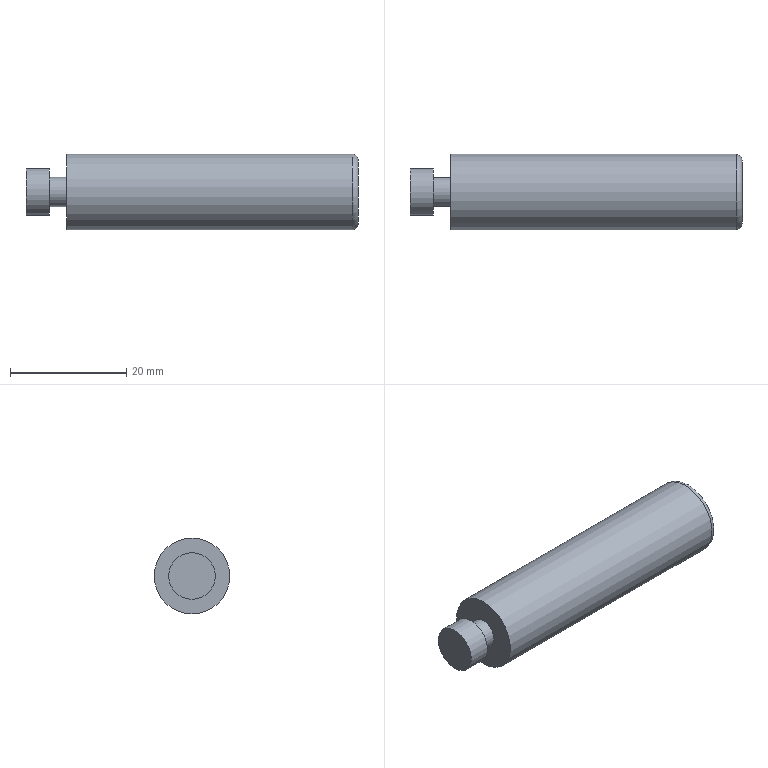Component | NX | SHAFT_02 | 1 solid | 8 faces | box 57 x 13 x 13 mm | volume 6888 mm3 | plane 4 | cylinder 3 | torus 1 | commonest cylinder face diameters 8 x1 5 x1 13 x1
STEP:
#1=CARTESIAN_POINT('',(0.,0.,0.));
#2=DIRECTION('',(0.,0.,1.));
#3=DIRECTION('',(1.,0.,0.));
#4=AXIS2_PLACEMENT_3D('',#1,#2,#3);
#5=CARTESIAN_POINT('',(100.,3.,1.5));
#6=VERTEX_POINT('',#5);
#7=CARTESIAN_POINT('',(100.,3.,4.));
#8=DIRECTION('',(1.,0.,0.));
#9=DIRECTION('',(0.,0.,-1.));
#10=AXIS2_PLACEMENT_3D('',#7,#8,#9);
#11=CIRCLE('',#10,2.5);
#12=CARTESIAN_POINT('',(100.,3.,4.));
#13=DIRECTION('',(1.,0.,0.));
#14=DIRECTION('',(0.,0.,-1.));
#15=AXIS2_PLACEMENT_3D('',#12,#13,#14);
#16=PLANE('',#15);
#17=CARTESIAN_POINT('',(0.,0.));
#18=DIRECTION('',(1.,0.));
#19=AXIS2_PLACEMENT_2D('',#17,#18);
#20=CIRCLE('',#19,2.5);
#21=(GEOMETRIC_REPRESENTATION_CONTEXT(2)PARAMETRIC_REPRESENTATION_CONTEXT()REPRESENTATION_CONTEXT('',''));
#22=DEFINITIONAL_REPRESENTATION('',(#20),#21);
#23=PCURVE('',#16,#22);
#24=CARTESIAN_POINT('',(100.,3.,4.));
#25=DIRECTION('',(1.,0.,0.));
#26=DIRECTION('',(0.,0.,-1.));
#27=AXIS2_PLACEMENT_3D('',#24,#25,#26);
#28=CYLINDRICAL_SURFACE('',#27,2.5);
#29=CARTESIAN_POINT('',(0.,0.));
#30=DIRECTION('',(1.,0.));
#31=VECTOR('',#30,1.);
#32=LINE('',#29,#31);
#33=(GEOMETRIC_REPRESENTATION_CONTEXT(2)PARAMETRIC_REPRESENTATION_CONTEXT()REPRESENTATION_CONTEXT('',''));
#34=DEFINITIONAL_REPRESENTATION('',(#32),#33);
#35=PCURVE('',#28,#34);
#36=SURFACE_CURVE('',#11,(#23,#35),.PCURVE_S1.);
#37=EDGE_CURVE('',#6,#6,#36,.T.);
#38=ORIENTED_EDGE('',*,*,#37,.F.);
#39=EDGE_LOOP('',(#38));
#40=FACE_BOUND('',#39,.T.);
#41=CARTESIAN_POINT('',(100.,3.,0.));
#42=VERTEX_POINT('',#41);
#43=CARTESIAN_POINT('',(100.,3.,4.));
#44=DIRECTION('',(-1.,0.,0.));
#45=DIRECTION('',(0.,0.,-1.));
#46=AXIS2_PLACEMENT_3D('',#43,#44,#45);
#47=CIRCLE('',#46,4.);
#48=CARTESIAN_POINT('',(4.,0.));
#49=CARTESIAN_POINT('',(4.,-6.928));
#50=CARTESIAN_POINT('',(-2.,-3.464));
#51=CARTESIAN_POINT('',(-8.,-0.));
#52=CARTESIAN_POINT('',(-2.,3.464));
#53=CARTESIAN_POINT('',(4.,6.928));
#54=CARTESIAN_POINT('',(4.,0.));
#55=(BOUNDED_CURVE()B_SPLINE_CURVE(2,(#48,#49,#50,#51,#52,#53,#54),.UNSPECIFIED.,.T.,.F.)B_SPLINE_CURVE_WITH_KNOTS((1,2,2,2,2,1),(-2.094,0.,2.094,4.189,6.283,8.378),.UNSPECIFIED.)CURVE()GEOMETRIC_REPRESENTATION_ITEM()RATIONAL_B_SPLINE_CURVE((1.,0.5,1.,0.5,1.,0.5,1.))REPRESENTATION_ITEM(''));
#56=(GEOMETRIC_REPRESENTATION_CONTEXT(2)PARAMETRIC_REPRESENTATION_CONTEXT()REPRESENTATION_CONTEXT('',''));
#57=DEFINITIONAL_REPRESENTATION('',(#55),#56);
#58=PCURVE('',#16,#57);
#59=CARTESIAN_POINT('',(96.,3.,4.));
#60=DIRECTION('',(1.,0.,0.));
#61=DIRECTION('',(0.,0.,-1.));
#62=AXIS2_PLACEMENT_3D('',#59,#60,#61);
#63=CYLINDRICAL_SURFACE('',#62,4.);
#64=CARTESIAN_POINT('',(6.283,4.));
#65=DIRECTION('',(-1.,0.));
#66=VECTOR('',#65,1.);
#67=LINE('',#64,#66);
#68=(GEOMETRIC_REPRESENTATION_CONTEXT(2)PARAMETRIC_REPRESENTATION_CONTEXT()REPRESENTATION_CONTEXT('',''));
#69=DEFINITIONAL_REPRESENTATION('',(#67),#68);
#70=PCURVE('',#63,#69);
#71=SURFACE_CURVE('',#47,(#58,#70),.PCURVE_S1.);
#72=EDGE_CURVE('',#42,#42,#71,.T.);
#73=ORIENTED_EDGE('',*,*,#72,.F.);
#74=EDGE_LOOP('',(#73));
#75=FACE_BOUND('',#74,.T.);
#76=ADVANCED_FACE('',(#40,#75),#16,.T.);
#77=CARTESIAN_POINT('',(96.,3.,0.));
#78=VERTEX_POINT('',#77);
#79=CARTESIAN_POINT('',(96.,3.,4.));
#80=DIRECTION('',(1.,0.,0.));
#81=DIRECTION('',(0.,0.,-1.));
#82=AXIS2_PLACEMENT_3D('',#79,#80,#81);
#83=CIRCLE('',#82,4.);
#84=CARTESIAN_POINT('',(96.,3.,4.));
#85=DIRECTION('',(-1.,0.,0.));
#86=DIRECTION('',(0.,0.,1.));
#87=AXIS2_PLACEMENT_3D('',#84,#85,#86);
#88=PLANE('',#87);
#89=CARTESIAN_POINT('',(-4.,0.));
#90=CARTESIAN_POINT('',(-4.,6.928));
#91=CARTESIAN_POINT('',(2.,3.464));
#92=CARTESIAN_POINT('',(8.,0.));
#93=CARTESIAN_POINT('',(2.,-3.464));
#94=CARTESIAN_POINT('',(-4.,-6.928));
#95=CARTESIAN_POINT('',(-4.,0.));
#96=(BOUNDED_CURVE()B_SPLINE_CURVE(2,(#89,#90,#91,#92,#93,#94,#95),.UNSPECIFIED.,.T.,.F.)B_SPLINE_CURVE_WITH_KNOTS((1,2,2,2,2,1),(-2.094,0.,2.094,4.189,6.283,8.378),.UNSPECIFIED.)CURVE()GEOMETRIC_REPRESENTATION_ITEM()RATIONAL_B_SPLINE_CURVE((1.,0.5,1.,0.5,1.,0.5,1.))REPRESENTATION_ITEM(''));
#97=(GEOMETRIC_REPRESENTATION_CONTEXT(2)PARAMETRIC_REPRESENTATION_CONTEXT()REPRESENTATION_CONTEXT('',''));
#98=DEFINITIONAL_REPRESENTATION('',(#96),#97);
#99=PCURVE('',#88,#98);
#100=CARTESIAN_POINT('',(0.,0.));
#101=DIRECTION('',(1.,0.));
#102=VECTOR('',#101,1.);
#103=LINE('',#100,#102);
#104=(GEOMETRIC_REPRESENTATION_CONTEXT(2)PARAMETRIC_REPRESENTATION_CONTEXT()REPRESENTATION_CONTEXT('',''));
#105=DEFINITIONAL_REPRESENTATION('',(#103),#104);
#106=PCURVE('',#63,#105);
#107=SURFACE_CURVE('',#83,(#99,#106),.PCURVE_S1.);
#108=EDGE_CURVE('',#78,#78,#107,.T.);
#109=ORIENTED_EDGE('',*,*,#108,.F.);
#110=EDGE_LOOP('',(#109));
#111=FACE_BOUND('',#110,.T.);
#112=ADVANCED_FACE('',(#111),#88,.T.);
#113=ORIENTED_EDGE('',*,*,#72,.T.);
#114=CARTESIAN_POINT('',(96.,3.,0.));
#115=CARTESIAN_POINT('',(100.,3.,0.));
#116=B_SPLINE_CURVE_WITH_KNOTS('',1,(#114,#115),.UNSPECIFIED.,.F.,.F.,(2,2),(0.,4.),.PIECEWISE_BEZIER_KNOTS.);
#117=CARTESIAN_POINT('',(0.,0.));
#118=DIRECTION('',(0.,1.));
#119=VECTOR('',#118,1.);
#120=LINE('',#117,#119);
#121=(GEOMETRIC_REPRESENTATION_CONTEXT(2)PARAMETRIC_REPRESENTATION_CONTEXT()REPRESENTATION_CONTEXT('',''));
#122=DEFINITIONAL_REPRESENTATION('',(#120),#121);
#123=PCURVE('',#63,#122);
#124=CARTESIAN_POINT('',(6.283,0.));
#125=DIRECTION('',(0.,1.));
#126=VECTOR('',#125,1.);
#127=LINE('',#124,#126);
#128=(GEOMETRIC_REPRESENTATION_CONTEXT(2)PARAMETRIC_REPRESENTATION_CONTEXT()REPRESENTATION_CONTEXT('',''));
#129=DEFINITIONAL_REPRESENTATION('',(#127),#128);
#130=PCURVE('',#63,#129);
#131=SEAM_CURVE('',#116,(#123,#130),.PCURVE_S1.);
#132=EDGE_CURVE('',#78,#42,#131,.T.);
#133=ORIENTED_EDGE('',*,*,#132,.F.);
#134=ORIENTED_EDGE('',*,*,#108,.T.);
#135=ORIENTED_EDGE('',*,*,#132,.T.);
#136=EDGE_LOOP('',(#113,#133,#134,#135));
#137=FACE_BOUND('',#136,.T.);
#138=ADVANCED_FACE('',(#137),#63,.T.);
#139=CARTESIAN_POINT('',(103.,3.,1.5));
#140=VERTEX_POINT('',#139);
#141=CARTESIAN_POINT('',(103.,3.,4.));
#142=DIRECTION('',(-1.,0.,0.));
#143=DIRECTION('',(0.,0.,-1.));
#144=AXIS2_PLACEMENT_3D('',#141,#142,#143);
#145=CIRCLE('',#144,2.5);
#146=CARTESIAN_POINT('',(6.283,3.));
#147=DIRECTION('',(-1.,0.));
#148=VECTOR('',#147,1.);
#149=LINE('',#146,#148);
#150=(GEOMETRIC_REPRESENTATION_CONTEXT(2)PARAMETRIC_REPRESENTATION_CONTEXT()REPRESENTATION_CONTEXT('',''));
#151=DEFINITIONAL_REPRESENTATION('',(#149),#150);
#152=PCURVE('',#28,#151);
#153=CARTESIAN_POINT('',(103.,3.,4.));
#154=DIRECTION('',(-1.,0.,0.));
#155=DIRECTION('',(0.,0.,1.));
#156=AXIS2_PLACEMENT_3D('',#153,#154,#155);
#157=PLANE('',#156);
#158=CARTESIAN_POINT('',(0.,0.));
#159=DIRECTION('',(-1.,0.));
#160=AXIS2_PLACEMENT_2D('',#158,#159);
#161=CIRCLE('',#160,2.5);
#162=(GEOMETRIC_REPRESENTATION_CONTEXT(2)PARAMETRIC_REPRESENTATION_CONTEXT()REPRESENTATION_CONTEXT('',''));
#163=DEFINITIONAL_REPRESENTATION('',(#161),#162);
#164=PCURVE('',#157,#163);
#165=SURFACE_CURVE('',#145,(#152,#164),.PCURVE_S1.);
#166=EDGE_CURVE('',#140,#140,#165,.T.);
#167=ORIENTED_EDGE('',*,*,#166,.T.);
#168=CARTESIAN_POINT('',(100.,3.,1.5));
#169=CARTESIAN_POINT('',(103.,3.,1.5));
#170=B_SPLINE_CURVE_WITH_KNOTS('',1,(#168,#169),.UNSPECIFIED.,.F.,.F.,(2,2),(0.,3.),.PIECEWISE_BEZIER_KNOTS.);
#171=CARTESIAN_POINT('',(0.,0.));
#172=DIRECTION('',(0.,1.));
#173=VECTOR('',#172,1.);
#174=LINE('',#171,#173);
#175=(GEOMETRIC_REPRESENTATION_CONTEXT(2)PARAMETRIC_REPRESENTATION_CONTEXT()REPRESENTATION_CONTEXT('',''));
#176=DEFINITIONAL_REPRESENTATION('',(#174),#175);
#177=PCURVE('',#28,#176);
#178=CARTESIAN_POINT('',(6.283,0.));
#179=DIRECTION('',(0.,1.));
#180=VECTOR('',#179,1.);
#181=LINE('',#178,#180);
#182=(GEOMETRIC_REPRESENTATION_CONTEXT(2)PARAMETRIC_REPRESENTATION_CONTEXT()REPRESENTATION_CONTEXT('',''));
#183=DEFINITIONAL_REPRESENTATION('',(#181),#182);
#184=PCURVE('',#28,#183);
#185=SEAM_CURVE('',#170,(#177,#184),.PCURVE_S1.);
#186=EDGE_CURVE('',#6,#140,#185,.T.);
#187=ORIENTED_EDGE('',*,*,#186,.F.);
#188=ORIENTED_EDGE('',*,*,#37,.T.);
#189=ORIENTED_EDGE('',*,*,#186,.T.);
#190=EDGE_LOOP('',(#167,#187,#188,#189));
#191=FACE_BOUND('',#190,.T.);
#192=ADVANCED_FACE('',(#191),#28,.T.);
#193=CARTESIAN_POINT('',(153.,3.,-1.5));
#194=VERTEX_POINT('',#193);
#195=CARTESIAN_POINT('',(153.,3.,4.));
#196=DIRECTION('',(1.,0.,0.));
#197=DIRECTION('',(0.,0.,-1.));
#198=AXIS2_PLACEMENT_3D('',#195,#196,#197);
#199=CIRCLE('',#198,5.5);
#200=CARTESIAN_POINT('',(153.,3.,4.));
#201=DIRECTION('',(1.,0.,0.));
#202=DIRECTION('',(0.,0.,-1.));
#203=AXIS2_PLACEMENT_3D('',#200,#201,#202);
#204=PLANE('',#203);
#205=CARTESIAN_POINT('',(0.,0.));
#206=DIRECTION('',(1.,0.));
#207=AXIS2_PLACEMENT_2D('',#205,#206);
#208=CIRCLE('',#207,5.5);
#209=(GEOMETRIC_REPRESENTATION_CONTEXT(2)PARAMETRIC_REPRESENTATION_CONTEXT()REPRESENTATION_CONTEXT('',''));
#210=DEFINITIONAL_REPRESENTATION('',(#208),#209);
#211=PCURVE('',#204,#210);
#212=CARTESIAN_POINT('',(152.,3.,4.));
#213=DIRECTION('',(1.,0.,0.));
#214=DIRECTION('',(0.,0.,-1.));
#215=AXIS2_PLACEMENT_3D('',#212,#213,#214);
#216=TOROIDAL_SURFACE('',#215,5.5,1.);
#217=CARTESIAN_POINT('',(0.,7.854));
#218=DIRECTION('',(1.,0.));
#219=VECTOR('',#218,1.);
#220=LINE('',#217,#219);
#221=(GEOMETRIC_REPRESENTATION_CONTEXT(2)PARAMETRIC_REPRESENTATION_CONTEXT()REPRESENTATION_CONTEXT('',''));
#222=DEFINITIONAL_REPRESENTATION('',(#220),#221);
#223=PCURVE('',#216,#222);
#224=SURFACE_CURVE('',#199,(#211,#223),.PCURVE_S1.);
#225=EDGE_CURVE('',#194,#194,#224,.T.);
#226=ORIENTED_EDGE('',*,*,#225,.T.);
#227=EDGE_LOOP('',(#226));
#228=FACE_BOUND('',#227,.T.);
#229=ADVANCED_FACE('',(#228),#204,.T.);
#230=ORIENTED_EDGE('',*,*,#166,.F.);
#231=EDGE_LOOP('',(#230));
#232=FACE_BOUND('',#231,.T.);
#233=CARTESIAN_POINT('',(103.,3.,-2.5));
#234=VERTEX_POINT('',#233);
#235=CARTESIAN_POINT('',(103.,3.,4.));
#236=DIRECTION('',(1.,0.,0.));
#237=DIRECTION('',(0.,0.,-1.));
#238=AXIS2_PLACEMENT_3D('',#235,#236,#237);
#239=CIRCLE('',#238,6.5);
#240=CARTESIAN_POINT('',(-6.5,0.));
#241=CARTESIAN_POINT('',(-6.5,11.258));
#242=CARTESIAN_POINT('',(3.25,5.629));
#243=CARTESIAN_POINT('',(13.,0.));
#244=CARTESIAN_POINT('',(3.25,-5.629));
#245=CARTESIAN_POINT('',(-6.5,-11.258));
#246=CARTESIAN_POINT('',(-6.5,0.));
#247=(BOUNDED_CURVE()B_SPLINE_CURVE(2,(#240,#241,#242,#243,#244,#245,#246),.UNSPECIFIED.,.T.,.F.)B_SPLINE_CURVE_WITH_KNOTS((1,2,2,2,2,1),(-2.094,0.,2.094,4.189,6.283,8.378),.UNSPECIFIED.)CURVE()GEOMETRIC_REPRESENTATION_ITEM()RATIONAL_B_SPLINE_CURVE((1.,0.5,1.,0.5,1.,0.5,1.))REPRESENTATION_ITEM(''));
#248=(GEOMETRIC_REPRESENTATION_CONTEXT(2)PARAMETRIC_REPRESENTATION_CONTEXT()REPRESENTATION_CONTEXT('',''));
#249=DEFINITIONAL_REPRESENTATION('',(#247),#248);
#250=PCURVE('',#157,#249);
#251=CARTESIAN_POINT('',(103.,3.,4.));
#252=DIRECTION('',(1.,0.,0.));
#253=DIRECTION('',(0.,0.,-1.));
#254=AXIS2_PLACEMENT_3D('',#251,#252,#253);
#255=CYLINDRICAL_SURFACE('',#254,6.5);
#256=CARTESIAN_POINT('',(0.,0.));
#257=DIRECTION('',(1.,0.));
#258=VECTOR('',#257,1.);
#259=LINE('',#256,#258);
#260=(GEOMETRIC_REPRESENTATION_CONTEXT(2)PARAMETRIC_REPRESENTATION_CONTEXT()REPRESENTATION_CONTEXT('',''));
#261=DEFINITIONAL_REPRESENTATION('',(#259),#260);
#262=PCURVE('',#255,#261);
#263=SURFACE_CURVE('',#239,(#250,#262),.PCURVE_S1.);
#264=EDGE_CURVE('',#234,#234,#263,.T.);
#265=ORIENTED_EDGE('',*,*,#264,.F.);
#266=EDGE_LOOP('',(#265));
#267=FACE_BOUND('',#266,.T.);
#268=ADVANCED_FACE('',(#232,#267),#157,.T.);
#269=CARTESIAN_POINT('',(152.,3.,-2.5));
#270=VERTEX_POINT('',#269);
#271=CARTESIAN_POINT('',(152.,3.,4.));
#272=DIRECTION('',(-1.,0.,0.));
#273=DIRECTION('',(0.,0.,-1.));
#274=AXIS2_PLACEMENT_3D('',#271,#272,#273);
#275=CIRCLE('',#274,6.5);
#276=CARTESIAN_POINT('',(6.283,49.));
#277=DIRECTION('',(-1.,0.));
#278=VECTOR('',#277,1.);
#279=LINE('',#276,#278);
#280=(GEOMETRIC_REPRESENTATION_CONTEXT(2)PARAMETRIC_REPRESENTATION_CONTEXT()REPRESENTATION_CONTEXT('',''));
#281=DEFINITIONAL_REPRESENTATION('',(#279),#280);
#282=PCURVE('',#255,#281);
#283=CARTESIAN_POINT('',(6.283,6.283));
#284=DIRECTION('',(-1.,0.));
#285=VECTOR('',#284,1.);
#286=LINE('',#283,#285);
#287=(GEOMETRIC_REPRESENTATION_CONTEXT(2)PARAMETRIC_REPRESENTATION_CONTEXT()REPRESENTATION_CONTEXT('',''));
#288=DEFINITIONAL_REPRESENTATION('',(#286),#287);
#289=PCURVE('',#216,#288);
#290=SURFACE_CURVE('',#275,(#282,#289),.PCURVE_S1.);
#291=EDGE_CURVE('',#270,#270,#290,.T.);
#292=ORIENTED_EDGE('',*,*,#291,.T.);
#293=CARTESIAN_POINT('',(103.,3.,-2.5));
#294=CARTESIAN_POINT('',(152.,3.,-2.5));
#295=B_SPLINE_CURVE_WITH_KNOTS('',1,(#293,#294),.UNSPECIFIED.,.F.,.F.,(2,2),(0.,49.),.PIECEWISE_BEZIER_KNOTS.);
#296=CARTESIAN_POINT('',(0.,0.));
#297=DIRECTION('',(0.,1.));
#298=VECTOR('',#297,1.);
#299=LINE('',#296,#298);
#300=(GEOMETRIC_REPRESENTATION_CONTEXT(2)PARAMETRIC_REPRESENTATION_CONTEXT()REPRESENTATION_CONTEXT('',''));
#301=DEFINITIONAL_REPRESENTATION('',(#299),#300);
#302=PCURVE('',#255,#301);
#303=CARTESIAN_POINT('',(6.283,0.));
#304=DIRECTION('',(0.,1.));
#305=VECTOR('',#304,1.);
#306=LINE('',#303,#305);
#307=(GEOMETRIC_REPRESENTATION_CONTEXT(2)PARAMETRIC_REPRESENTATION_CONTEXT()REPRESENTATION_CONTEXT('',''));
#308=DEFINITIONAL_REPRESENTATION('',(#306),#307);
#309=PCURVE('',#255,#308);
#310=SEAM_CURVE('',#295,(#302,#309),.PCURVE_S1.);
#311=EDGE_CURVE('',#234,#270,#310,.T.);
#312=ORIENTED_EDGE('',*,*,#311,.F.);
#313=ORIENTED_EDGE('',*,*,#264,.T.);
#314=ORIENTED_EDGE('',*,*,#311,.T.);
#315=EDGE_LOOP('',(#292,#312,#313,#314));
#316=FACE_BOUND('',#315,.T.);
#317=ADVANCED_FACE('',(#316),#255,.T.);
#318=ORIENTED_EDGE('',*,*,#225,.F.);
#319=CARTESIAN_POINT('',(152.,3.,-2.5));
#320=CARTESIAN_POINT('',(152.267,3.,-2.5));
#321=CARTESIAN_POINT('',(152.528,3.,-2.415));
#322=CARTESIAN_POINT('',(152.752,3.,-2.252));
#323=CARTESIAN_POINT('',(152.915,3.,-2.028));
#324=CARTESIAN_POINT('',(153.,3.,-1.767));
#325=CARTESIAN_POINT('',(153.,3.,-1.5));
#326=(BOUNDED_CURVE()B_SPLINE_CURVE(6,(#319,#320,#321,#322,#323,#324,#325),.UNSPECIFIED.,.F.,.F.)B_SPLINE_CURVE_WITH_KNOTS((7,7),(0.,1.571),.PIECEWISE_BEZIER_KNOTS.)CURVE()GEOMETRIC_REPRESENTATION_ITEM()RATIONAL_B_SPLINE_CURVE((1.031,1.01,0.9979,0.994,0.9979,1.01,1.031))REPRESENTATION_ITEM(''));
#327=CARTESIAN_POINT('',(0.,6.283));
#328=DIRECTION('',(0.,1.));
#329=VECTOR('',#328,1.);
#330=LINE('',#327,#329);
#331=(GEOMETRIC_REPRESENTATION_CONTEXT(2)PARAMETRIC_REPRESENTATION_CONTEXT()REPRESENTATION_CONTEXT('',''));
#332=DEFINITIONAL_REPRESENTATION('',(#330),#331);
#333=PCURVE('',#216,#332);
#334=CARTESIAN_POINT('',(6.283,6.283));
#335=DIRECTION('',(0.,1.));
#336=VECTOR('',#335,1.);
#337=LINE('',#334,#336);
#338=(GEOMETRIC_REPRESENTATION_CONTEXT(2)PARAMETRIC_REPRESENTATION_CONTEXT()REPRESENTATION_CONTEXT('',''));
#339=DEFINITIONAL_REPRESENTATION('',(#337),#338);
#340=PCURVE('',#216,#339);
#341=SEAM_CURVE('',#326,(#333,#340),.PCURVE_S1.);
#342=EDGE_CURVE('',#270,#194,#341,.T.);
#343=ORIENTED_EDGE('',*,*,#342,.F.);
#344=ORIENTED_EDGE('',*,*,#291,.F.);
#345=ORIENTED_EDGE('',*,*,#342,.T.);
#346=EDGE_LOOP('',(#318,#343,#344,#345));
#347=FACE_BOUND('',#346,.T.);
#348=ADVANCED_FACE('',(#347),#216,.T.);
#349=CLOSED_SHELL('',(#76,#112,#138,#192,#229,#268,#317,#348));
#350=MANIFOLD_SOLID_BREP('',#349);
#351=(LENGTH_UNIT()NAMED_UNIT(*)SI_UNIT(.MILLI.,.METRE.));
#352=UNCERTAINTY_MEASURE_WITH_UNIT(LENGTH_MEASURE(0.00001),#351,'','');
#353=(NAMED_UNIT(*)PLANE_ANGLE_UNIT()SI_UNIT($,.RADIAN.));
#354=(NAMED_UNIT(*)SI_UNIT($,.STERADIAN.)SOLID_ANGLE_UNIT());
#355=(GEOMETRIC_REPRESENTATION_CONTEXT(3)GLOBAL_UNCERTAINTY_ASSIGNED_CONTEXT((#352))GLOBAL_UNIT_ASSIGNED_CONTEXT((#351,#353,#354))REPRESENTATION_CONTEXT('',''));
#356=ADVANCED_BREP_SHAPE_REPRESENTATION('',(#4,#350),#355);